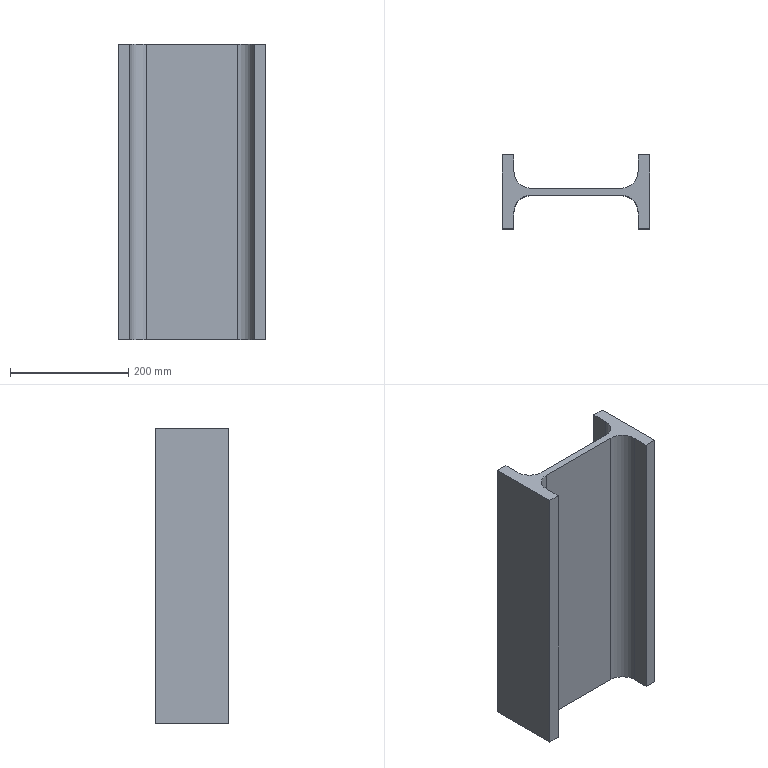Component | SolidWorks | Corbel-3 | 1 solid | 18 faces | box 250 x 125 x 500 mm | volume 4096496 mm3 | plane 14 | cylinder 4 | commonest cylinder face diameters 56 x4
build123d program:
from build123d import *

# Parameters (mm, degrees)
H_BEAM_HM600_300B_1_DEPTH = 500


with BuildPart() as part:
    # Sketch1 → H-Beam HM600_300B_1 (new body)
    with BuildSketch(Plane.YZ):
        with BuildLine():
            Line((-62.5, -125), (-62.5, -105))
            Line((-62.5, -105), (-34, -105))
            ThreePointArc((-34, -105), (-14.201, -96.799), (-6, -77))
            Line((-6, -77), (-6, 77))
            ThreePointArc((-6, 77), (-14.201, 96.799), (-34, 105))
            Line((-34, 105), (-62.5, 105))
            Line((-62.5, 105), (-62.5, 125))
            Line((-62.5, 125), (62.5, 125))
            Line((62.5, 125), (62.5, 105))
            Line((62.5, 105), (34, 105))
            ThreePointArc((34, 105), (14.201, 96.799), (6, 77))
            Line((6, 77), (6, -77))
            ThreePointArc((6, -77), (14.201, -96.799), (34, -105))
            Line((34, -105), (62.5, -105))
            Line((62.5, -105), (62.5, -125))
            Line((62.5, -125), (-62.5, -125))
        make_face()
    extrude(amount=H_BEAM_HM600_300B_1_DEPTH)


solid = part.part

# Placed as in the assembly
solid = solid.moved(Location((1694.926, -11132.346, 352.321), (0, 90, 0)))
STEP:
#1=COLOUR_RGB('',0.7922,0.8196,0.9333);
#2=FILL_AREA_STYLE_COLOUR('',#1);
#3=FILL_AREA_STYLE('',(#2));
#4=SURFACE_STYLE_FILL_AREA(#3);
#5=SURFACE_SIDE_STYLE('',(#4));
#6=SURFACE_STYLE_USAGE(.BOTH.,#5);
#7=PRESENTATION_STYLE_ASSIGNMENT((#6));
#8=CARTESIAN_POINT('',(71.651,-440.742,-5.814));
#9=VERTEX_POINT('',#8);
#10=CARTESIAN_POINT('',(71.651,-435.821,-5.814));
#11=VERTEX_POINT('',#10);
#12=CARTESIAN_POINT('',(71.651,-435.821,-5.814));
#13=DIRECTION('',(-0.,1.,-0.));
#14=VECTOR('',#13,39.37);
#15=LINE('',#12,#14);
#16=EDGE_CURVE('',#9,#11,#15,.T.);
#17=ORIENTED_EDGE('',*,*,#16,.T.);
#18=CARTESIAN_POINT('',(71.651,-435.821,13.871));
#19=VERTEX_POINT('',#18);
#20=CARTESIAN_POINT('',(71.651,-435.821,13.871));
#21=DIRECTION('',(-0.,-0.,-1.));
#22=VECTOR('',#21,39.37);
#23=LINE('',#20,#22);
#24=EDGE_CURVE('',#19,#11,#23,.T.);
#25=ORIENTED_EDGE('',*,*,#24,.F.);
#26=CARTESIAN_POINT('',(71.651,-440.742,13.871));
#27=VERTEX_POINT('',#26);
#28=CARTESIAN_POINT('',(71.651,-435.821,13.871));
#29=DIRECTION('',(-0.,1.,-0.));
#30=VECTOR('',#29,39.37);
#31=LINE('',#28,#30);
#32=EDGE_CURVE('',#27,#19,#31,.T.);
#33=ORIENTED_EDGE('',*,*,#32,.F.);
#34=CARTESIAN_POINT('',(71.651,-440.742,13.871));
#35=DIRECTION('',(-0.,-0.,-1.));
#36=VECTOR('',#35,39.37);
#37=LINE('',#34,#36);
#38=EDGE_CURVE('',#27,#9,#37,.T.);
#39=ORIENTED_EDGE('',*,*,#38,.T.);
#40=EDGE_LOOP('',(#17,#25,#33,#39));
#41=FACE_OUTER_BOUND('',#40,.T.);
#42=CARTESIAN_POINT('',(71.651,-435.821,13.871));
#43=DIRECTION('',(-1.,-0.,0.));
#44=DIRECTION('',(0.,0.,1.));
#45=AXIS2_PLACEMENT_3D('',#42,#43,#44);
#46=PLANE('',#45);
#47=ADVANCED_FACE('',(#41),#46,.F.);
#48=CARTESIAN_POINT('',(70.863,-435.821,-5.814));
#49=VERTEX_POINT('',#48);
#50=CARTESIAN_POINT('',(70.863,-435.821,-5.814));
#51=DIRECTION('',(-1.,-0.,0.));
#52=VECTOR('',#51,39.37);
#53=LINE('',#50,#52);
#54=EDGE_CURVE('',#11,#49,#53,.T.);
#55=ORIENTED_EDGE('',*,*,#54,.T.);
#56=CARTESIAN_POINT('',(70.863,-435.821,13.871));
#57=VERTEX_POINT('',#56);
#58=CARTESIAN_POINT('',(70.863,-435.821,13.871));
#59=DIRECTION('',(-0.,-0.,-1.));
#60=VECTOR('',#59,39.37);
#61=LINE('',#58,#60);
#62=EDGE_CURVE('',#57,#49,#61,.T.);
#63=ORIENTED_EDGE('',*,*,#62,.F.);
#64=CARTESIAN_POINT('',(70.863,-435.821,13.871));
#65=DIRECTION('',(-1.,-0.,0.));
#66=VECTOR('',#65,39.37);
#67=LINE('',#64,#66);
#68=EDGE_CURVE('',#19,#57,#67,.T.);
#69=ORIENTED_EDGE('',*,*,#68,.F.);
#70=ORIENTED_EDGE('',*,*,#24,.T.);
#71=EDGE_LOOP('',(#55,#63,#69,#70));
#72=FACE_OUTER_BOUND('',#71,.T.);
#73=CARTESIAN_POINT('',(70.863,-435.821,13.871));
#74=DIRECTION('',(0.,-1.,0.));
#75=DIRECTION('',(1.,0.,-0.));
#76=AXIS2_PLACEMENT_3D('',#73,#74,#75);
#77=PLANE('',#76);
#78=ADVANCED_FACE('',(#72),#77,.F.);
#79=CARTESIAN_POINT('',(70.863,-436.943,-5.814));
#80=VERTEX_POINT('',#79);
#81=CARTESIAN_POINT('',(70.863,-435.821,-5.814));
#82=DIRECTION('',(-0.,-1.,0.));
#83=VECTOR('',#82,39.37);
#84=LINE('',#81,#83);
#85=EDGE_CURVE('',#49,#80,#84,.T.);
#86=ORIENTED_EDGE('',*,*,#85,.T.);
#87=CARTESIAN_POINT('',(70.863,-436.943,13.871));
#88=VERTEX_POINT('',#87);
#89=CARTESIAN_POINT('',(70.863,-436.943,13.871));
#90=DIRECTION('',(-0.,-0.,-1.));
#91=VECTOR('',#90,39.37);
#92=LINE('',#89,#91);
#93=EDGE_CURVE('',#88,#80,#92,.T.);
#94=ORIENTED_EDGE('',*,*,#93,.F.);
#95=CARTESIAN_POINT('',(70.863,-435.821,13.871));
#96=DIRECTION('',(-0.,-1.,0.));
#97=VECTOR('',#96,39.37);
#98=LINE('',#95,#97);
#99=EDGE_CURVE('',#57,#88,#98,.T.);
#100=ORIENTED_EDGE('',*,*,#99,.F.);
#101=ORIENTED_EDGE('',*,*,#62,.T.);
#102=EDGE_LOOP('',(#86,#94,#100,#101));
#103=FACE_OUTER_BOUND('',#102,.T.);
#104=CARTESIAN_POINT('',(70.863,-435.821,13.871));
#105=DIRECTION('',(1.,-0.,-0.));
#106=DIRECTION('',(0.,1.,-0.));
#107=AXIS2_PLACEMENT_3D('',#104,#105,#106);
#108=PLANE('',#107);
#109=ADVANCED_FACE('',(#103),#108,.F.);
#110=CARTESIAN_POINT('',(69.761,-438.045,-5.814));
#111=VERTEX_POINT('',#110);
#112=CARTESIAN_POINT('',(69.761,-436.943,-5.814));
#113=DIRECTION('',(-0.,-0.,-1.));
#114=DIRECTION('',(-1.,0.,0.));
#115=AXIS2_PLACEMENT_3D('',#112,#113,#114);
#116=CIRCLE('',#115,1.102);
#117=EDGE_CURVE('',#80,#111,#116,.T.);
#118=ORIENTED_EDGE('',*,*,#117,.T.);
#119=CARTESIAN_POINT('',(69.761,-438.045,13.871));
#120=VERTEX_POINT('',#119);
#121=CARTESIAN_POINT('',(69.761,-438.045,13.871));
#122=DIRECTION('',(-0.,-0.,-1.));
#123=VECTOR('',#122,39.37);
#124=LINE('',#121,#123);
#125=EDGE_CURVE('',#120,#111,#124,.T.);
#126=ORIENTED_EDGE('',*,*,#125,.F.);
#127=CARTESIAN_POINT('',(69.761,-436.943,13.871));
#128=DIRECTION('',(-0.,-0.,-1.));
#129=DIRECTION('',(-1.,0.,0.));
#130=AXIS2_PLACEMENT_3D('',#127,#128,#129);
#131=CIRCLE('',#130,1.102);
#132=EDGE_CURVE('',#88,#120,#131,.T.);
#133=ORIENTED_EDGE('',*,*,#132,.F.);
#134=ORIENTED_EDGE('',*,*,#93,.T.);
#135=EDGE_LOOP('',(#118,#126,#133,#134));
#136=FACE_OUTER_BOUND('',#135,.T.);
#137=CARTESIAN_POINT('',(69.761,-436.943,13.871));
#138=DIRECTION('',(-0.,-0.,-1.));
#139=DIRECTION('',(-1.,0.,0.));
#140=AXIS2_PLACEMENT_3D('',#137,#138,#139);
#141=CYLINDRICAL_SURFACE('',#140,1.102);
#142=ADVANCED_FACE('',(#136),#141,.F.);
#143=CARTESIAN_POINT('',(63.698,-438.045,-5.814));
#144=VERTEX_POINT('',#143);
#145=CARTESIAN_POINT('',(63.698,-438.045,-5.814));
#146=DIRECTION('',(-1.,-0.,0.));
#147=VECTOR('',#146,39.37);
#148=LINE('',#145,#147);
#149=EDGE_CURVE('',#111,#144,#148,.T.);
#150=ORIENTED_EDGE('',*,*,#149,.T.);
#151=CARTESIAN_POINT('',(63.698,-438.045,13.871));
#152=VERTEX_POINT('',#151);
#153=CARTESIAN_POINT('',(63.698,-438.045,13.871));
#154=DIRECTION('',(-0.,-0.,-1.));
#155=VECTOR('',#154,39.37);
#156=LINE('',#153,#155);
#157=EDGE_CURVE('',#152,#144,#156,.T.);
#158=ORIENTED_EDGE('',*,*,#157,.F.);
#159=CARTESIAN_POINT('',(63.698,-438.045,13.871));
#160=DIRECTION('',(-1.,-0.,0.));
#161=VECTOR('',#160,39.37);
#162=LINE('',#159,#161);
#163=EDGE_CURVE('',#120,#152,#162,.T.);
#164=ORIENTED_EDGE('',*,*,#163,.F.);
#165=ORIENTED_EDGE('',*,*,#125,.T.);
#166=EDGE_LOOP('',(#150,#158,#164,#165));
#167=FACE_OUTER_BOUND('',#166,.T.);
#168=CARTESIAN_POINT('',(63.698,-438.045,13.871));
#169=DIRECTION('',(0.,-1.,0.));
#170=DIRECTION('',(1.,0.,-0.));
#171=AXIS2_PLACEMENT_3D('',#168,#169,#170);
#172=PLANE('',#171);
#173=ADVANCED_FACE('',(#167),#172,.F.);
#174=CARTESIAN_POINT('',(62.596,-436.943,-5.814));
#175=VERTEX_POINT('',#174);
#176=CARTESIAN_POINT('',(63.698,-436.943,-5.814));
#177=DIRECTION('',(-0.,-0.,-1.));
#178=DIRECTION('',(-1.,0.,0.));
#179=AXIS2_PLACEMENT_3D('',#176,#177,#178);
#180=CIRCLE('',#179,1.102);
#181=EDGE_CURVE('',#144,#175,#180,.T.);
#182=ORIENTED_EDGE('',*,*,#181,.T.);
#183=CARTESIAN_POINT('',(62.596,-436.943,13.871));
#184=VERTEX_POINT('',#183);
#185=CARTESIAN_POINT('',(62.596,-436.943,13.871));
#186=DIRECTION('',(-0.,-0.,-1.));
#187=VECTOR('',#186,39.37);
#188=LINE('',#185,#187);
#189=EDGE_CURVE('',#184,#175,#188,.T.);
#190=ORIENTED_EDGE('',*,*,#189,.F.);
#191=CARTESIAN_POINT('',(63.698,-436.943,13.871));
#192=DIRECTION('',(-0.,-0.,-1.));
#193=DIRECTION('',(-1.,0.,0.));
#194=AXIS2_PLACEMENT_3D('',#191,#192,#193);
#195=CIRCLE('',#194,1.102);
#196=EDGE_CURVE('',#152,#184,#195,.T.);
#197=ORIENTED_EDGE('',*,*,#196,.F.);
#198=ORIENTED_EDGE('',*,*,#157,.T.);
#199=EDGE_LOOP('',(#182,#190,#197,#198));
#200=FACE_OUTER_BOUND('',#199,.T.);
#201=CARTESIAN_POINT('',(63.698,-436.943,13.871));
#202=DIRECTION('',(-0.,-0.,-1.));
#203=DIRECTION('',(-1.,0.,0.));
#204=AXIS2_PLACEMENT_3D('',#201,#202,#203);
#205=CYLINDRICAL_SURFACE('',#204,1.102);
#206=ADVANCED_FACE('',(#200),#205,.F.);
#207=CARTESIAN_POINT('',(62.596,-435.821,-5.814));
#208=VERTEX_POINT('',#207);
#209=CARTESIAN_POINT('',(62.596,-436.943,-5.814));
#210=DIRECTION('',(0.,1.,-0.));
#211=VECTOR('',#210,39.37);
#212=LINE('',#209,#211);
#213=EDGE_CURVE('',#175,#208,#212,.T.);
#214=ORIENTED_EDGE('',*,*,#213,.T.);
#215=CARTESIAN_POINT('',(62.596,-435.821,13.871));
#216=VERTEX_POINT('',#215);
#217=CARTESIAN_POINT('',(62.596,-435.821,13.871));
#218=DIRECTION('',(-0.,-0.,-1.));
#219=VECTOR('',#218,39.37);
#220=LINE('',#217,#219);
#221=EDGE_CURVE('',#216,#208,#220,.T.);
#222=ORIENTED_EDGE('',*,*,#221,.F.);
#223=CARTESIAN_POINT('',(62.596,-436.943,13.871));
#224=DIRECTION('',(0.,1.,-0.));
#225=VECTOR('',#224,39.37);
#226=LINE('',#223,#225);
#227=EDGE_CURVE('',#184,#216,#226,.T.);
#228=ORIENTED_EDGE('',*,*,#227,.F.);
#229=ORIENTED_EDGE('',*,*,#189,.T.);
#230=EDGE_LOOP('',(#214,#222,#228,#229));
#231=FACE_OUTER_BOUND('',#230,.T.);
#232=CARTESIAN_POINT('',(62.596,-436.943,13.871));
#233=DIRECTION('',(-1.,0.,0.));
#234=DIRECTION('',(-0.,-1.,0.));
#235=AXIS2_PLACEMENT_3D('',#232,#233,#234);
#236=PLANE('',#235);
#237=ADVANCED_FACE('',(#231),#236,.F.);
#238=CARTESIAN_POINT('',(61.808,-435.821,-5.814));
#239=VERTEX_POINT('',#238);
#240=CARTESIAN_POINT('',(61.808,-435.821,-5.814));
#241=DIRECTION('',(-1.,-0.,0.));
#242=VECTOR('',#241,39.37);
#243=LINE('',#240,#242);
#244=EDGE_CURVE('',#208,#239,#243,.T.);
#245=ORIENTED_EDGE('',*,*,#244,.T.);
#246=CARTESIAN_POINT('',(61.808,-435.821,13.871));
#247=VERTEX_POINT('',#246);
#248=CARTESIAN_POINT('',(61.808,-435.821,13.871));
#249=DIRECTION('',(-0.,-0.,-1.));
#250=VECTOR('',#249,39.37);
#251=LINE('',#248,#250);
#252=EDGE_CURVE('',#247,#239,#251,.T.);
#253=ORIENTED_EDGE('',*,*,#252,.F.);
#254=CARTESIAN_POINT('',(61.808,-435.821,13.871));
#255=DIRECTION('',(-1.,-0.,0.));
#256=VECTOR('',#255,39.37);
#257=LINE('',#254,#256);
#258=EDGE_CURVE('',#216,#247,#257,.T.);
#259=ORIENTED_EDGE('',*,*,#258,.F.);
#260=ORIENTED_EDGE('',*,*,#221,.T.);
#261=EDGE_LOOP('',(#245,#253,#259,#260));
#262=FACE_OUTER_BOUND('',#261,.T.);
#263=CARTESIAN_POINT('',(61.808,-435.821,13.871));
#264=DIRECTION('',(0.,-1.,0.));
#265=DIRECTION('',(1.,0.,-0.));
#266=AXIS2_PLACEMENT_3D('',#263,#264,#265);
#267=PLANE('',#266);
#268=ADVANCED_FACE('',(#262),#267,.F.);
#269=CARTESIAN_POINT('',(61.808,-440.742,-5.814));
#270=VERTEX_POINT('',#269);
#271=CARTESIAN_POINT('',(61.808,-440.742,-5.814));
#272=DIRECTION('',(0.,-1.,0.));
#273=VECTOR('',#272,39.37);
#274=LINE('',#271,#273);
#275=EDGE_CURVE('',#239,#270,#274,.T.);
#276=ORIENTED_EDGE('',*,*,#275,.T.);
#277=CARTESIAN_POINT('',(61.808,-440.742,13.871));
#278=VERTEX_POINT('',#277);
#279=CARTESIAN_POINT('',(61.808,-440.742,13.871));
#280=DIRECTION('',(-0.,-0.,-1.));
#281=VECTOR('',#280,39.37);
#282=LINE('',#279,#281);
#283=EDGE_CURVE('',#278,#270,#282,.T.);
#284=ORIENTED_EDGE('',*,*,#283,.F.);
#285=CARTESIAN_POINT('',(61.808,-440.742,13.871));
#286=DIRECTION('',(0.,-1.,0.));
#287=VECTOR('',#286,39.37);
#288=LINE('',#285,#287);
#289=EDGE_CURVE('',#247,#278,#288,.T.);
#290=ORIENTED_EDGE('',*,*,#289,.F.);
#291=ORIENTED_EDGE('',*,*,#252,.T.);
#292=EDGE_LOOP('',(#276,#284,#290,#291));
#293=FACE_OUTER_BOUND('',#292,.T.);
#294=CARTESIAN_POINT('',(61.808,-440.742,13.871));
#295=DIRECTION('',(1.,0.,-0.));
#296=DIRECTION('',(-0.,-0.,-1.));
#297=AXIS2_PLACEMENT_3D('',#294,#295,#296);
#298=PLANE('',#297);
#299=ADVANCED_FACE('',(#293),#298,.F.);
#300=CARTESIAN_POINT('',(62.596,-440.742,-5.814));
#301=VERTEX_POINT('',#300);
#302=CARTESIAN_POINT('',(62.596,-440.742,-5.814));
#303=DIRECTION('',(1.,0.,-0.));
#304=VECTOR('',#303,39.37);
#305=LINE('',#302,#304);
#306=EDGE_CURVE('',#270,#301,#305,.T.);
#307=ORIENTED_EDGE('',*,*,#306,.T.);
#308=CARTESIAN_POINT('',(62.596,-440.742,13.871));
#309=VERTEX_POINT('',#308);
#310=CARTESIAN_POINT('',(62.596,-440.742,13.871));
#311=DIRECTION('',(-0.,-0.,-1.));
#312=VECTOR('',#311,39.37);
#313=LINE('',#310,#312);
#314=EDGE_CURVE('',#309,#301,#313,.T.);
#315=ORIENTED_EDGE('',*,*,#314,.F.);
#316=CARTESIAN_POINT('',(62.596,-440.742,13.871));
#317=DIRECTION('',(1.,0.,-0.));
#318=VECTOR('',#317,39.37);
#319=LINE('',#316,#318);
#320=EDGE_CURVE('',#278,#309,#319,.T.);
#321=ORIENTED_EDGE('',*,*,#320,.F.);
#322=ORIENTED_EDGE('',*,*,#283,.T.);
#323=EDGE_LOOP('',(#307,#315,#321,#322));
#324=FACE_OUTER_BOUND('',#323,.T.);
#325=CARTESIAN_POINT('',(62.596,-440.742,13.871));
#326=DIRECTION('',(-0.,1.,-0.));
#327=DIRECTION('',(-1.,-0.,0.));
#328=AXIS2_PLACEMENT_3D('',#325,#326,#327);
#329=PLANE('',#328);
#330=ADVANCED_FACE('',(#324),#329,.F.);
#331=CARTESIAN_POINT('',(62.596,-439.62,-5.814));
#332=VERTEX_POINT('',#331);
#333=CARTESIAN_POINT('',(62.596,-440.742,-5.814));
#334=DIRECTION('',(-0.,1.,-0.));
#335=VECTOR('',#334,39.37);
#336=LINE('',#333,#335);
#337=EDGE_CURVE('',#301,#332,#336,.T.);
#338=ORIENTED_EDGE('',*,*,#337,.T.);
#339=CARTESIAN_POINT('',(62.596,-439.62,13.871));
#340=VERTEX_POINT('',#339);
#341=CARTESIAN_POINT('',(62.596,-439.62,13.871));
#342=DIRECTION('',(-0.,-0.,-1.));
#343=VECTOR('',#342,39.37);
#344=LINE('',#341,#343);
#345=EDGE_CURVE('',#340,#332,#344,.T.);
#346=ORIENTED_EDGE('',*,*,#345,.F.);
#347=CARTESIAN_POINT('',(62.596,-440.742,13.871));
#348=DIRECTION('',(-0.,1.,-0.));
#349=VECTOR('',#348,39.37);
#350=LINE('',#347,#349);
#351=EDGE_CURVE('',#309,#340,#350,.T.);
#352=ORIENTED_EDGE('',*,*,#351,.F.);
#353=ORIENTED_EDGE('',*,*,#314,.T.);
#354=EDGE_LOOP('',(#338,#346,#352,#353));
#355=FACE_OUTER_BOUND('',#354,.T.);
#356=CARTESIAN_POINT('',(62.596,-440.742,13.871));
#357=DIRECTION('',(-1.,-0.,0.));
#358=DIRECTION('',(0.,-1.,0.));
#359=AXIS2_PLACEMENT_3D('',#356,#357,#358);
#360=PLANE('',#359);
#361=ADVANCED_FACE('',(#355),#360,.F.);
#362=CARTESIAN_POINT('',(63.698,-438.518,-5.814));
#363=VERTEX_POINT('',#362);
#364=CARTESIAN_POINT('',(63.698,-439.62,-5.814));
#365=DIRECTION('',(-0.,-0.,-1.));
#366=DIRECTION('',(1.,0.,0.));
#367=AXIS2_PLACEMENT_3D('',#364,#365,#366);
#368=CIRCLE('',#367,1.102);
#369=EDGE_CURVE('',#332,#363,#368,.T.);
#370=ORIENTED_EDGE('',*,*,#369,.T.);
#371=CARTESIAN_POINT('',(63.698,-438.518,13.871));
#372=VERTEX_POINT('',#371);
#373=CARTESIAN_POINT('',(63.698,-438.518,13.871));
#374=DIRECTION('',(-0.,-0.,-1.));
#375=VECTOR('',#374,39.37);
#376=LINE('',#373,#375);
#377=EDGE_CURVE('',#372,#363,#376,.T.);
#378=ORIENTED_EDGE('',*,*,#377,.F.);
#379=CARTESIAN_POINT('',(63.698,-439.62,13.871));
#380=DIRECTION('',(-0.,-0.,-1.));
#381=DIRECTION('',(1.,0.,0.));
#382=AXIS2_PLACEMENT_3D('',#379,#380,#381);
#383=CIRCLE('',#382,1.102);
#384=EDGE_CURVE('',#340,#372,#383,.T.);
#385=ORIENTED_EDGE('',*,*,#384,.F.);
#386=ORIENTED_EDGE('',*,*,#345,.T.);
#387=EDGE_LOOP('',(#370,#378,#385,#386));
#388=FACE_OUTER_BOUND('',#387,.T.);
#389=CARTESIAN_POINT('',(63.698,-439.62,13.871));
#390=DIRECTION('',(-0.,-0.,-1.));
#391=DIRECTION('',(-1.,0.,0.));
#392=AXIS2_PLACEMENT_3D('',#389,#390,#391);
#393=CYLINDRICAL_SURFACE('',#392,1.102);
#394=ADVANCED_FACE('',(#388),#393,.F.);
#395=CARTESIAN_POINT('',(69.761,-438.518,-5.814));
#396=VERTEX_POINT('',#395);
#397=CARTESIAN_POINT('',(69.761,-438.518,-5.814));
#398=DIRECTION('',(1.,0.,-0.));
#399=VECTOR('',#398,39.37);
#400=LINE('',#397,#399);
#401=EDGE_CURVE('',#363,#396,#400,.T.);
#402=ORIENTED_EDGE('',*,*,#401,.T.);
#403=CARTESIAN_POINT('',(69.761,-438.518,13.871));
#404=VERTEX_POINT('',#403);
#405=CARTESIAN_POINT('',(69.761,-438.518,13.871));
#406=DIRECTION('',(-0.,-0.,-1.));
#407=VECTOR('',#406,39.37);
#408=LINE('',#405,#407);
#409=EDGE_CURVE('',#404,#396,#408,.T.);
#410=ORIENTED_EDGE('',*,*,#409,.F.);
#411=CARTESIAN_POINT('',(69.761,-438.518,13.871));
#412=DIRECTION('',(1.,0.,-0.));
#413=VECTOR('',#412,39.37);
#414=LINE('',#411,#413);
#415=EDGE_CURVE('',#372,#404,#414,.T.);
#416=ORIENTED_EDGE('',*,*,#415,.F.);
#417=ORIENTED_EDGE('',*,*,#377,.T.);
#418=EDGE_LOOP('',(#402,#410,#416,#417));
#419=FACE_OUTER_BOUND('',#418,.T.);
#420=CARTESIAN_POINT('',(69.761,-438.518,13.871));
#421=DIRECTION('',(-0.,1.,-0.));
#422=DIRECTION('',(-1.,-0.,0.));
#423=AXIS2_PLACEMENT_3D('',#420,#421,#422);
#424=PLANE('',#423);
#425=ADVANCED_FACE('',(#419),#424,.F.);
#426=CARTESIAN_POINT('',(70.863,-439.62,-5.814));
#427=VERTEX_POINT('',#426);
#428=CARTESIAN_POINT('',(69.761,-439.62,-5.814));
#429=DIRECTION('',(-0.,-0.,-1.));
#430=DIRECTION('',(1.,0.,0.));
#431=AXIS2_PLACEMENT_3D('',#428,#429,#430);
#432=CIRCLE('',#431,1.102);
#433=EDGE_CURVE('',#396,#427,#432,.T.);
#434=ORIENTED_EDGE('',*,*,#433,.T.);
#435=CARTESIAN_POINT('',(70.863,-439.62,13.871));
#436=VERTEX_POINT('',#435);
#437=CARTESIAN_POINT('',(70.863,-439.62,13.871));
#438=DIRECTION('',(-0.,-0.,-1.));
#439=VECTOR('',#438,39.37);
#440=LINE('',#437,#439);
#441=EDGE_CURVE('',#436,#427,#440,.T.);
#442=ORIENTED_EDGE('',*,*,#441,.F.);
#443=CARTESIAN_POINT('',(69.761,-439.62,13.871));
#444=DIRECTION('',(-0.,-0.,-1.));
#445=DIRECTION('',(1.,0.,0.));
#446=AXIS2_PLACEMENT_3D('',#443,#444,#445);
#447=CIRCLE('',#446,1.102);
#448=EDGE_CURVE('',#404,#436,#447,.T.);
#449=ORIENTED_EDGE('',*,*,#448,.F.);
#450=ORIENTED_EDGE('',*,*,#409,.T.);
#451=EDGE_LOOP('',(#434,#442,#449,#450));
#452=FACE_OUTER_BOUND('',#451,.T.);
#453=CARTESIAN_POINT('',(69.761,-439.62,13.871));
#454=DIRECTION('',(-0.,-0.,-1.));
#455=DIRECTION('',(-1.,0.,0.));
#456=AXIS2_PLACEMENT_3D('',#453,#454,#455);
#457=CYLINDRICAL_SURFACE('',#456,1.102);
#458=ADVANCED_FACE('',(#452),#457,.F.);
#459=CARTESIAN_POINT('',(70.863,-440.742,-5.814));
#460=VERTEX_POINT('',#459);
#461=CARTESIAN_POINT('',(70.863,-439.62,-5.814));
#462=DIRECTION('',(0.,-1.,0.));
#463=VECTOR('',#462,39.37);
#464=LINE('',#461,#463);
#465=EDGE_CURVE('',#427,#460,#464,.T.);
#466=ORIENTED_EDGE('',*,*,#465,.T.);
#467=CARTESIAN_POINT('',(70.863,-440.742,13.871));
#468=VERTEX_POINT('',#467);
#469=CARTESIAN_POINT('',(70.863,-440.742,13.871));
#470=DIRECTION('',(-0.,-0.,-1.));
#471=VECTOR('',#470,39.37);
#472=LINE('',#469,#471);
#473=EDGE_CURVE('',#468,#460,#472,.T.);
#474=ORIENTED_EDGE('',*,*,#473,.F.);
#475=CARTESIAN_POINT('',(70.863,-439.62,13.871));
#476=DIRECTION('',(0.,-1.,0.));
#477=VECTOR('',#476,39.37);
#478=LINE('',#475,#477);
#479=EDGE_CURVE('',#436,#468,#478,.T.);
#480=ORIENTED_EDGE('',*,*,#479,.F.);
#481=ORIENTED_EDGE('',*,*,#441,.T.);
#482=EDGE_LOOP('',(#466,#474,#480,#481));
#483=FACE_OUTER_BOUND('',#482,.T.);
#484=CARTESIAN_POINT('',(70.863,-439.62,13.871));
#485=DIRECTION('',(1.,0.,-0.));
#486=DIRECTION('',(-0.,-0.,-1.));
#487=AXIS2_PLACEMENT_3D('',#484,#485,#486);
#488=PLANE('',#487);
#489=ADVANCED_FACE('',(#483),#488,.F.);
#490=CARTESIAN_POINT('',(71.651,-440.742,-5.814));
#491=DIRECTION('',(1.,0.,-0.));
#492=VECTOR('',#491,39.37);
#493=LINE('',#490,#492);
#494=EDGE_CURVE('',#460,#9,#493,.T.);
#495=ORIENTED_EDGE('',*,*,#494,.T.);
#496=ORIENTED_EDGE('',*,*,#38,.F.);
#497=CARTESIAN_POINT('',(71.651,-440.742,13.871));
#498=DIRECTION('',(1.,0.,-0.));
#499=VECTOR('',#498,39.37);
#500=LINE('',#497,#499);
#501=EDGE_CURVE('',#468,#27,#500,.T.);
#502=ORIENTED_EDGE('',*,*,#501,.F.);
#503=ORIENTED_EDGE('',*,*,#473,.T.);
#504=EDGE_LOOP('',(#495,#496,#502,#503));
#505=FACE_OUTER_BOUND('',#504,.T.);
#506=CARTESIAN_POINT('',(71.651,-440.742,13.871));
#507=DIRECTION('',(-0.,1.,-0.));
#508=DIRECTION('',(-1.,-0.,0.));
#509=AXIS2_PLACEMENT_3D('',#506,#507,#508);
#510=PLANE('',#509);
#511=ADVANCED_FACE('',(#505),#510,.F.);
#512=ORIENTED_EDGE('',*,*,#32,.T.);
#513=ORIENTED_EDGE('',*,*,#68,.T.);
#514=ORIENTED_EDGE('',*,*,#99,.T.);
#515=ORIENTED_EDGE('',*,*,#132,.T.);
#516=ORIENTED_EDGE('',*,*,#163,.T.);
#517=ORIENTED_EDGE('',*,*,#196,.T.);
#518=ORIENTED_EDGE('',*,*,#227,.T.);
#519=ORIENTED_EDGE('',*,*,#258,.T.);
#520=ORIENTED_EDGE('',*,*,#289,.T.);
#521=ORIENTED_EDGE('',*,*,#320,.T.);
#522=ORIENTED_EDGE('',*,*,#351,.T.);
#523=ORIENTED_EDGE('',*,*,#384,.T.);
#524=ORIENTED_EDGE('',*,*,#415,.T.);
#525=ORIENTED_EDGE('',*,*,#448,.T.);
#526=ORIENTED_EDGE('',*,*,#479,.T.);
#527=ORIENTED_EDGE('',*,*,#501,.T.);
#528=EDGE_LOOP('',(#512,#513,#514,#515,#516,#517,#518,#519,#520,#521,#522,#523,#524,#525,#526,#527));
#529=FACE_OUTER_BOUND('',#528,.T.);
#530=CARTESIAN_POINT('',(69.761,-439.62,13.871));
#531=DIRECTION('',(0.,0.,1.));
#532=DIRECTION('',(1.,0.,-0.));
#533=AXIS2_PLACEMENT_3D('',#530,#531,#532);
#534=PLANE('',#533);
#535=ADVANCED_FACE('',(#529),#534,.T.);
#536=ORIENTED_EDGE('',*,*,#16,.F.);
#537=ORIENTED_EDGE('',*,*,#494,.F.);
#538=ORIENTED_EDGE('',*,*,#465,.F.);
#539=ORIENTED_EDGE('',*,*,#433,.F.);
#540=ORIENTED_EDGE('',*,*,#401,.F.);
#541=ORIENTED_EDGE('',*,*,#369,.F.);
#542=ORIENTED_EDGE('',*,*,#337,.F.);
#543=ORIENTED_EDGE('',*,*,#306,.F.);
#544=ORIENTED_EDGE('',*,*,#275,.F.);
#545=ORIENTED_EDGE('',*,*,#244,.F.);
#546=ORIENTED_EDGE('',*,*,#213,.F.);
#547=ORIENTED_EDGE('',*,*,#181,.F.);
#548=ORIENTED_EDGE('',*,*,#149,.F.);
#549=ORIENTED_EDGE('',*,*,#117,.F.);
#550=ORIENTED_EDGE('',*,*,#85,.F.);
#551=ORIENTED_EDGE('',*,*,#54,.F.);
#552=EDGE_LOOP('',(#536,#537,#538,#539,#540,#541,#542,#543,#544,#545,#546,#547,#548,#549,#550,#551));
#553=FACE_OUTER_BOUND('',#552,.T.);
#554=CARTESIAN_POINT('',(69.761,-439.62,-5.814));
#555=DIRECTION('',(0.,0.,1.));
#556=DIRECTION('',(1.,0.,-0.));
#557=AXIS2_PLACEMENT_3D('',#554,#555,#556);
#558=PLANE('',#557);
#559=ADVANCED_FACE('',(#553),#558,.F.);
#560=CLOSED_SHELL('',(#47,#78,#109,#142,#173,#206,#237,#268,#299,#330,#361,#394,#425,#458,#489,#511,#535,#559));
#561=MANIFOLD_SOLID_BREP('',#560);
#562=STYLED_ITEM('',(#7),#561);
#563=PRESENTATION_LAYER_ASSIGNMENT('','',(#562));
#564=CARTESIAN_POINT('',(0.,0.,0.));
#565=DIRECTION('',(0.,0.,1.));
#566=DIRECTION('',(1.,0.,0.));
#567=AXIS2_PLACEMENT_3D('',#564,#565,#566);
#568=(LENGTH_UNIT()NAMED_UNIT(*)SI_UNIT($,.METRE.));
#569=LENGTH_MEASURE_WITH_UNIT(LENGTH_MEASURE(0.0254),#568);
#570=DIMENSIONAL_EXPONENTS(1.,0.,0.,0.,0.,0.,0.);
#571=(CONVERSION_BASED_UNIT('',#569)LENGTH_UNIT()NAMED_UNIT(#570));
#572=UNCERTAINTY_MEASURE_WITH_UNIT(LENGTH_MEASURE(0.00001),#571,'','');
#573=(NAMED_UNIT(*)PLANE_ANGLE_UNIT()SI_UNIT($,.RADIAN.));
#574=(NAMED_UNIT(*)SI_UNIT($,.STERADIAN.)SOLID_ANGLE_UNIT());
#575=(GEOMETRIC_REPRESENTATION_CONTEXT(3)GLOBAL_UNCERTAINTY_ASSIGNED_CONTEXT((#572))GLOBAL_UNIT_ASSIGNED_CONTEXT((#571,#573,#574))REPRESENTATION_CONTEXT('',''));
#576=ADVANCED_BREP_SHAPE_REPRESENTATION('',(#561,#567),#575);
#577=(LENGTH_UNIT()NAMED_UNIT(*)SI_UNIT($,.METRE.));
#578=LENGTH_MEASURE_WITH_UNIT(LENGTH_MEASURE(0.0254),#577);
#579=DIMENSIONAL_EXPONENTS(1.,0.,0.,0.,0.,0.,0.);
#580=(CONVERSION_BASED_UNIT('',#578)LENGTH_UNIT()NAMED_UNIT(#579));
#581=UNCERTAINTY_MEASURE_WITH_UNIT(LENGTH_MEASURE(0.00001),#580,'','');
#582=(NAMED_UNIT(*)PLANE_ANGLE_UNIT()SI_UNIT($,.RADIAN.));
#583=(NAMED_UNIT(*)SI_UNIT($,.STERADIAN.)SOLID_ANGLE_UNIT());
#584=(GEOMETRIC_REPRESENTATION_CONTEXT(3)GLOBAL_UNCERTAINTY_ASSIGNED_CONTEXT((#581))GLOBAL_UNIT_ASSIGNED_CONTEXT((#580,#582,#583))REPRESENTATION_CONTEXT('',''));
#585=MECHANICAL_DESIGN_GEOMETRIC_PRESENTATION_REPRESENTATION('',(#562),#584);